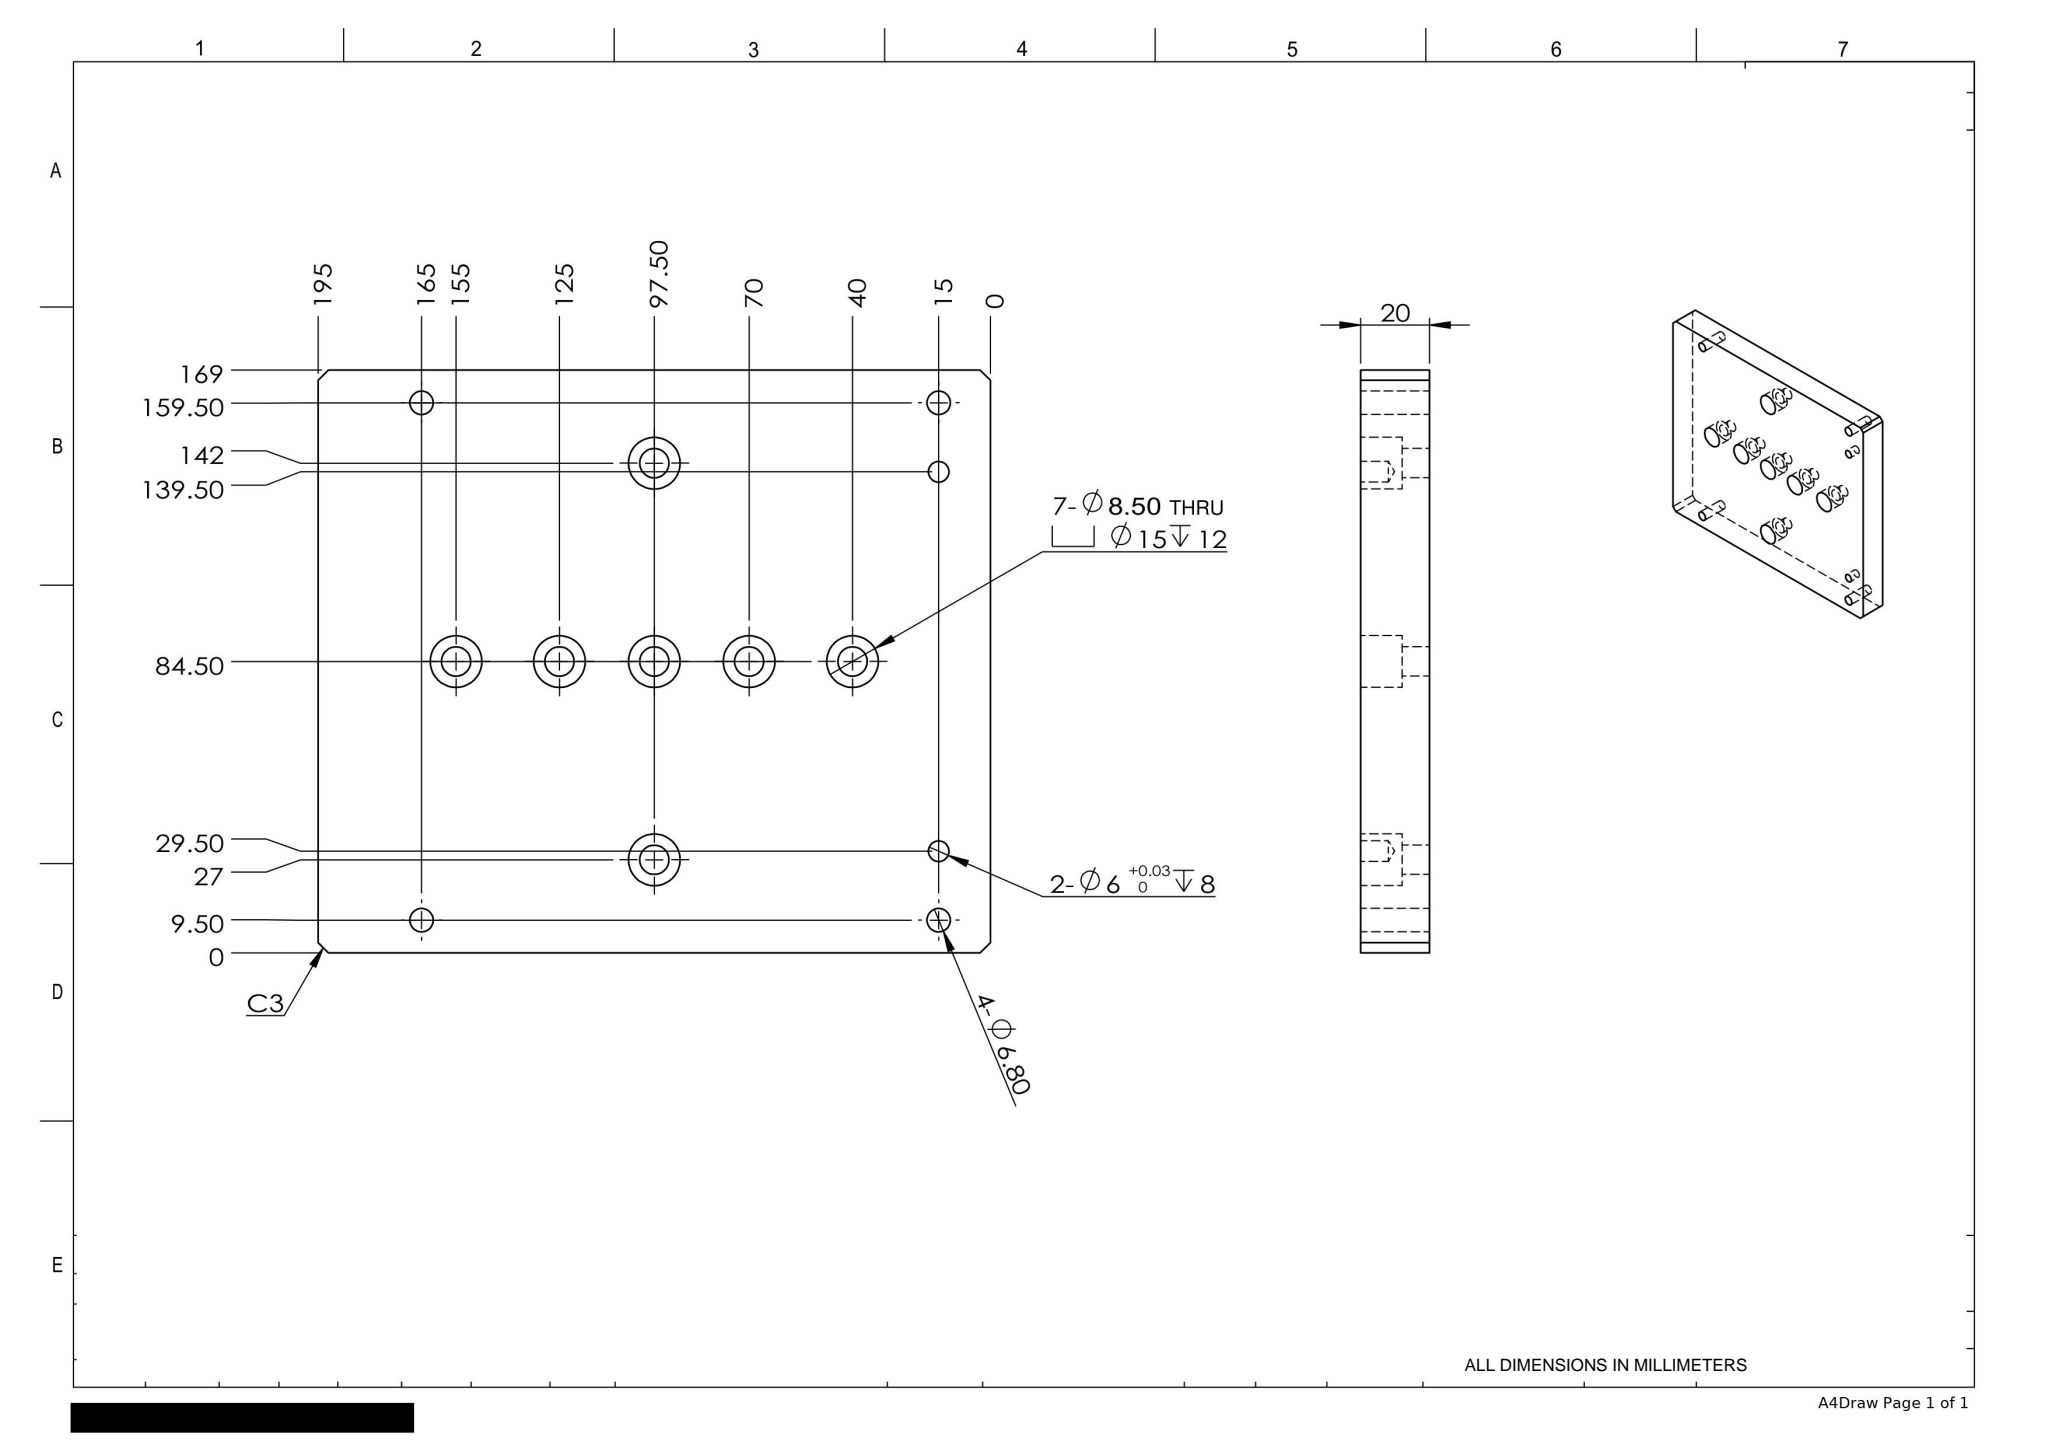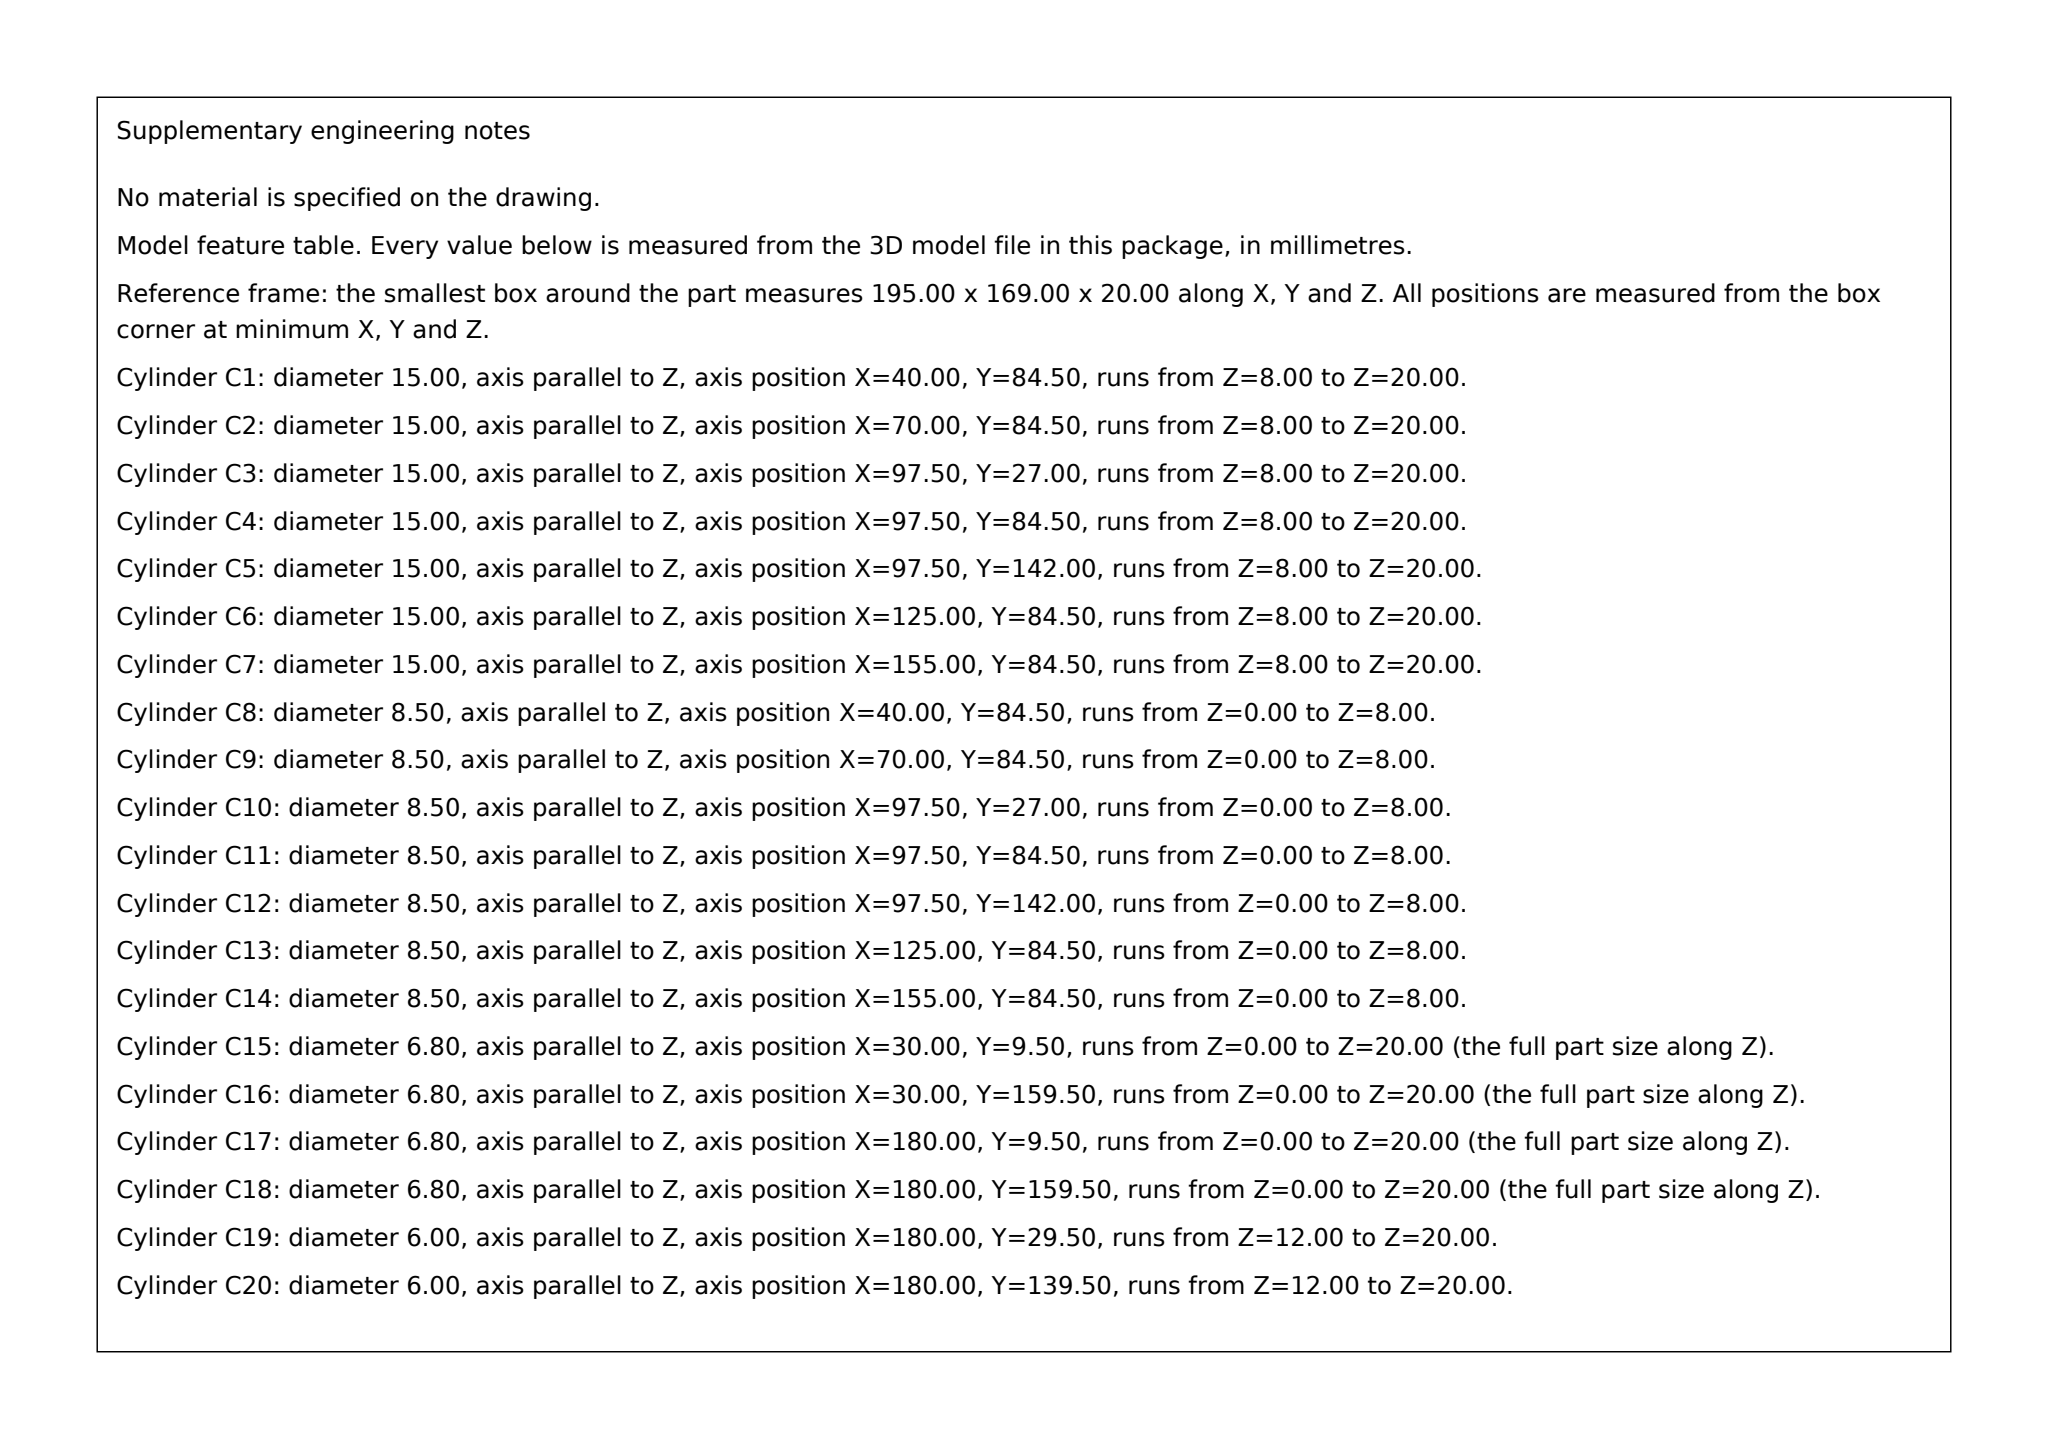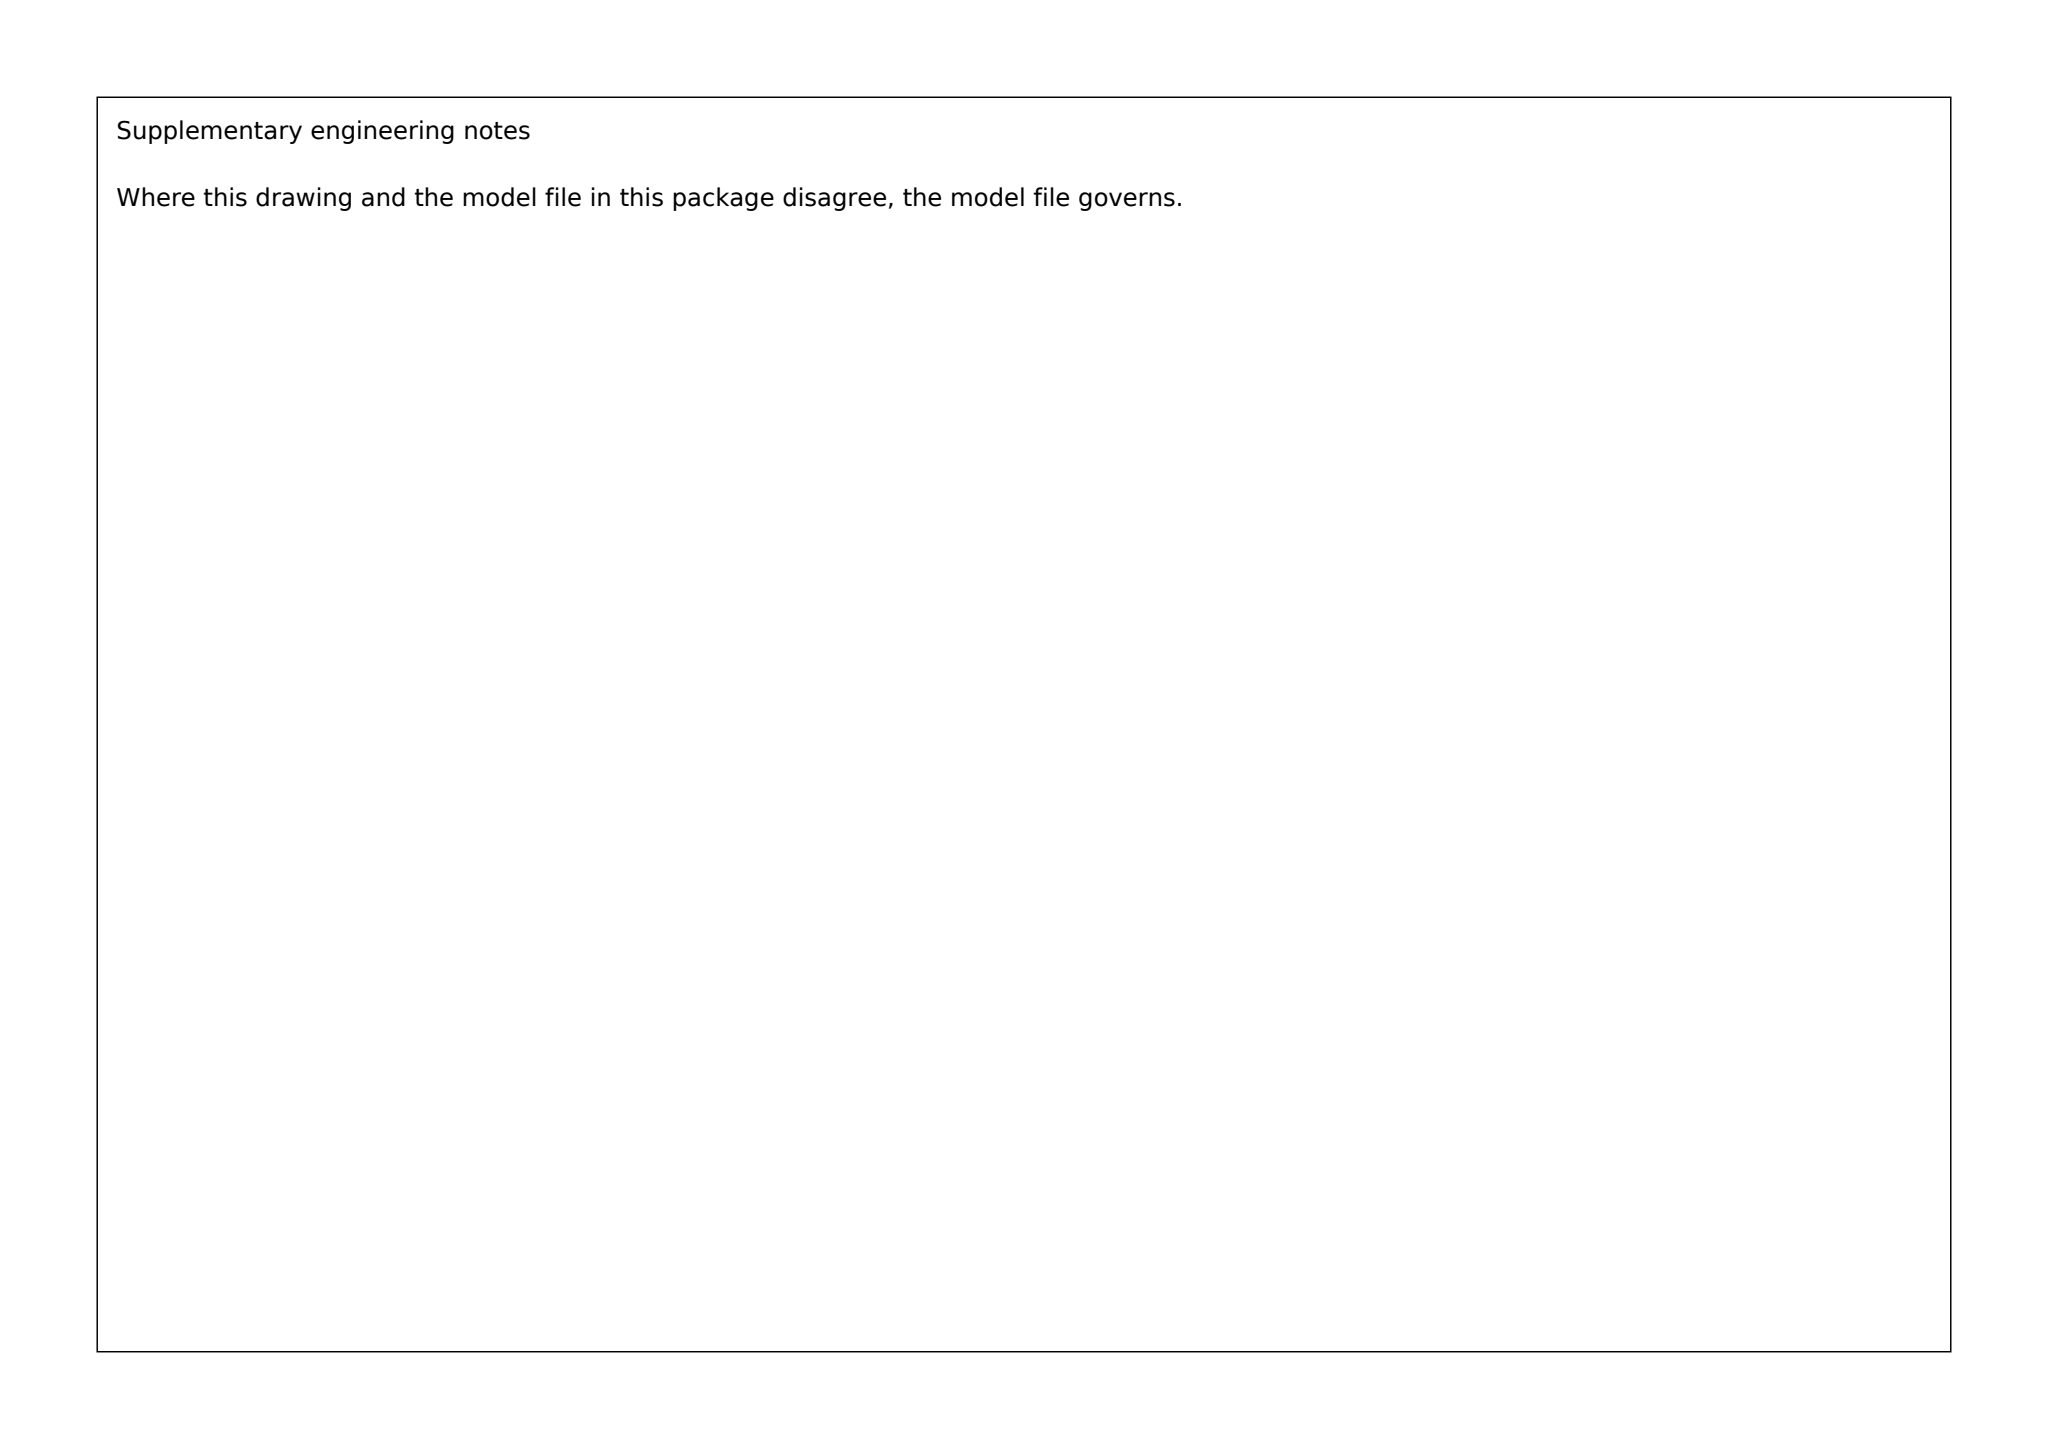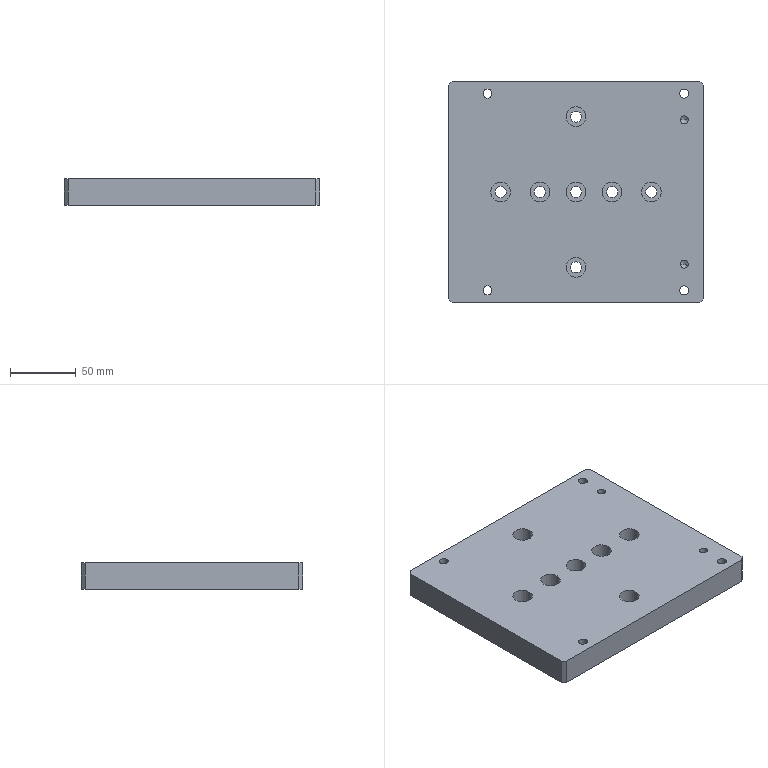Part | SolidWorks | mm | 1 solid | 61 faces | box 195 x 169 x 20 mm | volume 637327 mm3 | cylinder 40 | plane 17 | cone 4 | commonest cylinder face diameters 8.5 x14 15 x14 6.8 x8 6 x4